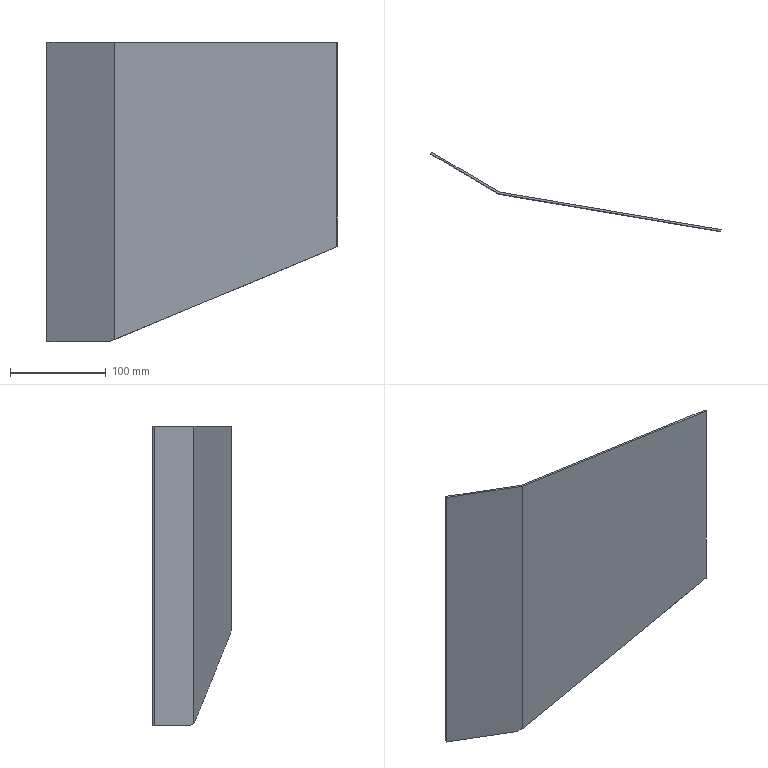Component | SolidWorks | LeftMaterialInletPlate-1 | 1 solid | 11 faces | box 303.24 x 82.86 x 313 mm | volume 174651 mm3 | plane 11
STEP:
#1=COLOUR_RGB('',0.7922,0.8196,0.9333);
#2=FILL_AREA_STYLE_COLOUR('',#1);
#3=FILL_AREA_STYLE('',(#2));
#4=SURFACE_STYLE_FILL_AREA(#3);
#5=SURFACE_SIDE_STYLE('',(#4));
#6=SURFACE_STYLE_USAGE(.BOTH.,#5);
#7=PRESENTATION_STYLE_ASSIGNMENT((#6));
#8=CARTESIAN_POINT('',(-3.729,-25.956,-0.4535));
#9=VERTEX_POINT('',#8);
#10=CARTESIAN_POINT('',(-3.731,-25.969,-0.4535));
#11=VERTEX_POINT('',#10);
#12=CARTESIAN_POINT('',(-3.667,-25.59,-0.4535));
#13=DIRECTION('',(-0.1671,-0.9859,-0.));
#14=VECTOR('',#13,39.37);
#15=LINE('',#12,#14);
#16=EDGE_CURVE('',#9,#11,#15,.T.);
#17=ORIENTED_EDGE('',*,*,#16,.F.);
#18=CARTESIAN_POINT('',(-3.543,-25.989,-0.3759));
#19=VERTEX_POINT('',#18);
#20=CARTESIAN_POINT('',(5.621,-27.645,3.443));
#21=DIRECTION('',(0.9105,-0.1645,0.3794));
#22=VECTOR('',#21,39.37);
#23=LINE('',#20,#22);
#24=EDGE_CURVE('',#9,#19,#23,.T.);
#25=ORIENTED_EDGE('',*,*,#24,.T.);
#26=CARTESIAN_POINT('',(-3.495,-26.018,-0.3543));
#27=VERTEX_POINT('',#26);
#28=CARTESIAN_POINT('',(-3.064,-26.273,-0.163));
#29=DIRECTION('',(-0.8037,0.4756,-0.3576));
#30=VECTOR('',#29,39.37);
#31=LINE('',#28,#30);
#32=EDGE_CURVE('',#27,#19,#31,.T.);
#33=ORIENTED_EDGE('',*,*,#32,.F.);
#34=CARTESIAN_POINT('',(-1.706,-26.321,0.3897));
#35=VERTEX_POINT('',#34);
#36=CARTESIAN_POINT('',(-6.771,-25.463,-1.717));
#37=DIRECTION('',(0.9122,-0.1546,0.3795));
#38=VECTOR('',#37,39.37);
#39=LINE('',#36,#38);
#40=EDGE_CURVE('',#27,#35,#39,.T.);
#41=ORIENTED_EDGE('',*,*,#40,.T.);
#42=CARTESIAN_POINT('',(5.454,-27.615,3.373));
#43=VERTEX_POINT('',#42);
#44=CARTESIAN_POINT('',(5.621,-27.645,3.443));
#45=DIRECTION('',(0.9105,-0.1645,0.3794));
#46=VECTOR('',#45,39.37);
#47=LINE('',#44,#46);
#48=EDGE_CURVE('',#35,#43,#47,.T.);
#49=ORIENTED_EDGE('',*,*,#48,.T.);
#50=CARTESIAN_POINT('',(-3.522,-26.093,-0.3603));
#51=VERTEX_POINT('',#50);
#52=CARTESIAN_POINT('',(-6.784,-25.541,-1.717));
#53=DIRECTION('',(0.9122,-0.1546,0.3795));
#54=VECTOR('',#53,39.37);
#55=LINE('',#52,#54);
#56=EDGE_CURVE('',#51,#43,#55,.T.);
#57=ORIENTED_EDGE('',*,*,#56,.F.);
#58=CARTESIAN_POINT('',(-3.101,-26.342,-0.1731));
#59=DIRECTION('',(-0.8037,0.4756,-0.3576));
#60=VECTOR('',#59,39.37);
#61=LINE('',#58,#60);
#62=EDGE_CURVE('',#51,#11,#61,.T.);
#63=ORIENTED_EDGE('',*,*,#62,.T.);
#64=EDGE_LOOP('',(#17,#25,#33,#41,#49,#57,#63));
#65=FACE_OUTER_BOUND('',#64,.T.);
#66=CARTESIAN_POINT('',(5.704,-27.178,3.445));
#67=DIRECTION('',(0.3741,-0.0634,-0.9252));
#68=DIRECTION('',(-0.8037,0.4756,-0.3576));
#69=AXIS2_PLACEMENT_3D('',#66,#67,#68);
#70=PLANE('',#69);
#71=ADVANCED_FACE('',(#65),#70,.T.);
#72=CARTESIAN_POINT('',(-3.837,-25.815,-0.4535));
#73=VERTEX_POINT('',#72);
#74=CARTESIAN_POINT('',(-5.432,-23.744,-0.4535));
#75=DIRECTION('',(-0.61,0.7924,0.));
#76=VECTOR('',#75,39.37);
#77=LINE('',#74,#76);
#78=EDGE_CURVE('',#9,#73,#77,.T.);
#79=ORIENTED_EDGE('',*,*,#78,.F.);
#80=ORIENTED_EDGE('',*,*,#16,.T.);
#81=CARTESIAN_POINT('',(-6.3,-24.449,-0.4535));
#82=VERTEX_POINT('',#81);
#83=CARTESIAN_POINT('',(-6.3,-24.449,-0.4535));
#84=DIRECTION('',(-0.8606,0.5093,0.));
#85=VECTOR('',#84,39.37);
#86=LINE('',#83,#85);
#87=EDGE_CURVE('',#11,#82,#86,.T.);
#88=ORIENTED_EDGE('',*,*,#87,.T.);
#89=CARTESIAN_POINT('',(-6.26,-24.381,-0.4535));
#90=VERTEX_POINT('',#89);
#91=CARTESIAN_POINT('',(-6.26,-24.381,-0.4535));
#92=DIRECTION('',(-0.5093,-0.8606,-0.));
#93=VECTOR('',#92,39.37);
#94=LINE('',#91,#93);
#95=EDGE_CURVE('',#90,#82,#94,.T.);
#96=ORIENTED_EDGE('',*,*,#95,.F.);
#97=CARTESIAN_POINT('',(-6.26,-24.381,-0.4535));
#98=DIRECTION('',(-0.8606,0.5093,0.));
#99=VECTOR('',#98,39.37);
#100=LINE('',#97,#99);
#101=EDGE_CURVE('',#73,#90,#100,.T.);
#102=ORIENTED_EDGE('',*,*,#101,.F.);
#103=EDGE_LOOP('',(#79,#80,#88,#96,#102));
#104=FACE_OUTER_BOUND('',#103,.T.);
#105=CARTESIAN_POINT('',(-6.26,-24.381,-0.4535));
#106=DIRECTION('',(-0.,0.,1.));
#107=DIRECTION('',(-0.5093,-0.8606,-0.));
#108=AXIS2_PLACEMENT_3D('',#105,#106,#107);
#109=PLANE('',#108);
#110=ADVANCED_FACE('',(#104),#109,.F.);
#111=CARTESIAN_POINT('',(5.638,-27.566,3.481));
#112=VERTEX_POINT('',#111);
#113=CARTESIAN_POINT('',(5.625,-27.644,3.446));
#114=VERTEX_POINT('',#113);
#115=CARTESIAN_POINT('',(4.811,-32.448,1.261));
#116=DIRECTION('',(-0.1525,-0.8997,-0.4091));
#117=VECTOR('',#116,39.37);
#118=LINE('',#115,#117);
#119=EDGE_CURVE('',#112,#114,#118,.T.);
#120=ORIENTED_EDGE('',*,*,#119,.F.);
#121=CARTESIAN_POINT('',(5.638,-27.566,11.869));
#122=VERTEX_POINT('',#121);
#123=CARTESIAN_POINT('',(5.638,-27.566,-9.784));
#124=DIRECTION('',(0.,0.,1.));
#125=VECTOR('',#124,39.37);
#126=LINE('',#123,#125);
#127=EDGE_CURVE('',#112,#122,#126,.T.);
#128=ORIENTED_EDGE('',*,*,#127,.T.);
#129=CARTESIAN_POINT('',(5.625,-27.644,11.869));
#130=VERTEX_POINT('',#129);
#131=CARTESIAN_POINT('',(5.638,-27.566,11.869));
#132=DIRECTION('',(-0.1671,-0.9859,-0.));
#133=VECTOR('',#132,39.37);
#134=LINE('',#131,#133);
#135=EDGE_CURVE('',#122,#130,#134,.T.);
#136=ORIENTED_EDGE('',*,*,#135,.T.);
#137=CARTESIAN_POINT('',(5.625,-27.644,-9.784));
#138=DIRECTION('',(0.,0.,1.));
#139=VECTOR('',#138,39.37);
#140=LINE('',#137,#139);
#141=EDGE_CURVE('',#114,#130,#140,.T.);
#142=ORIENTED_EDGE('',*,*,#141,.F.);
#143=EDGE_LOOP('',(#120,#128,#136,#142));
#144=FACE_OUTER_BOUND('',#143,.T.);
#145=CARTESIAN_POINT('',(5.638,-27.566,-9.784));
#146=DIRECTION('',(-0.9859,0.1671,0.));
#147=DIRECTION('',(0.1671,0.9859,0.));
#148=AXIS2_PLACEMENT_3D('',#145,#146,#147);
#149=PLANE('',#148);
#150=ADVANCED_FACE('',(#144),#149,.F.);
#151=ORIENTED_EDGE('',*,*,#127,.F.);
#152=CARTESIAN_POINT('',(-6.795,-25.459,-1.752));
#153=DIRECTION('',(0.9106,-0.1543,0.3833));
#154=VECTOR('',#153,39.37);
#155=LINE('',#152,#154);
#156=EDGE_CURVE('',#35,#112,#155,.T.);
#157=ORIENTED_EDGE('',*,*,#156,.F.);
#158=ORIENTED_EDGE('',*,*,#40,.F.);
#159=CARTESIAN_POINT('',(-3.495,-26.018,11.869));
#160=VERTEX_POINT('',#159);
#161=CARTESIAN_POINT('',(-3.495,-26.018,1.063));
#162=DIRECTION('',(0.,-0.,-1.));
#163=VECTOR('',#162,39.37);
#164=LINE('',#161,#163);
#165=EDGE_CURVE('',#160,#27,#164,.T.);
#166=ORIENTED_EDGE('',*,*,#165,.F.);
#167=CARTESIAN_POINT('',(-3.509,-26.016,11.869));
#168=DIRECTION('',(0.9859,-0.1671,-0.));
#169=VECTOR('',#168,39.37);
#170=LINE('',#167,#169);
#171=EDGE_CURVE('',#160,#122,#170,.T.);
#172=ORIENTED_EDGE('',*,*,#171,.T.);
#173=EDGE_LOOP('',(#151,#157,#158,#166,#172));
#174=FACE_OUTER_BOUND('',#173,.T.);
#175=CARTESIAN_POINT('',(-3.509,-26.016,-9.784));
#176=DIRECTION('',(-0.1671,-0.9859,-0.));
#177=DIRECTION('',(-0.9859,0.1671,0.));
#178=AXIS2_PLACEMENT_3D('',#175,#176,#177);
#179=PLANE('',#178);
#180=ADVANCED_FACE('',(#174),#179,.F.);
#181=ORIENTED_EDGE('',*,*,#32,.T.);
#182=CARTESIAN_POINT('',(-3.205,-26.19,-0.2869));
#183=DIRECTION('',(-0.8393,0.4967,-0.2211));
#184=VECTOR('',#183,39.37);
#185=LINE('',#182,#184);
#186=EDGE_CURVE('',#19,#73,#185,.T.);
#187=ORIENTED_EDGE('',*,*,#186,.T.);
#188=ORIENTED_EDGE('',*,*,#101,.T.);
#189=CARTESIAN_POINT('',(-6.26,-24.381,11.869));
#190=VERTEX_POINT('',#189);
#191=CARTESIAN_POINT('',(-6.26,-24.381,-0.4535));
#192=DIRECTION('',(0.,-0.,1.));
#193=VECTOR('',#192,39.37);
#194=LINE('',#191,#193);
#195=EDGE_CURVE('',#90,#190,#194,.T.);
#196=ORIENTED_EDGE('',*,*,#195,.T.);
#197=CARTESIAN_POINT('',(-6.26,-24.381,11.869));
#198=DIRECTION('',(0.8606,-0.5093,-0.));
#199=VECTOR('',#198,39.37);
#200=LINE('',#197,#199);
#201=EDGE_CURVE('',#190,#160,#200,.T.);
#202=ORIENTED_EDGE('',*,*,#201,.T.);
#203=ORIENTED_EDGE('',*,*,#165,.T.);
#204=EDGE_LOOP('',(#181,#187,#188,#196,#202,#203));
#205=FACE_OUTER_BOUND('',#204,.T.);
#206=CARTESIAN_POINT('',(-3.468,-26.034,1.063));
#207=DIRECTION('',(0.5093,0.8606,0.));
#208=DIRECTION('',(0.8606,-0.5093,-0.));
#209=AXIS2_PLACEMENT_3D('',#206,#207,#208);
#210=PLANE('',#209);
#211=ADVANCED_FACE('',(#205),#210,.T.);
#212=ORIENTED_EDGE('',*,*,#56,.T.);
#213=CARTESIAN_POINT('',(-6.796,-25.539,-1.782));
#214=DIRECTION('',(0.9106,-0.1543,0.3833));
#215=VECTOR('',#214,39.37);
#216=LINE('',#213,#215);
#217=EDGE_CURVE('',#43,#114,#216,.T.);
#218=ORIENTED_EDGE('',*,*,#217,.T.);
#219=ORIENTED_EDGE('',*,*,#141,.T.);
#220=CARTESIAN_POINT('',(-3.522,-26.093,11.869));
#221=VERTEX_POINT('',#220);
#222=CARTESIAN_POINT('',(-3.522,-26.093,11.869));
#223=DIRECTION('',(0.9859,-0.1671,-0.));
#224=VECTOR('',#223,39.37);
#225=LINE('',#222,#224);
#226=EDGE_CURVE('',#221,#130,#225,.T.);
#227=ORIENTED_EDGE('',*,*,#226,.F.);
#228=CARTESIAN_POINT('',(-3.522,-26.093,-0.4535));
#229=DIRECTION('',(-0.,0.,-1.));
#230=VECTOR('',#229,39.37);
#231=LINE('',#228,#230);
#232=EDGE_CURVE('',#221,#51,#231,.T.);
#233=ORIENTED_EDGE('',*,*,#232,.T.);
#234=EDGE_LOOP('',(#212,#218,#219,#227,#233));
#235=FACE_OUTER_BOUND('',#234,.T.);
#236=CARTESIAN_POINT('',(-3.522,-26.093,-9.784));
#237=DIRECTION('',(-0.1671,-0.9859,-0.));
#238=DIRECTION('',(-0.9859,0.1671,0.));
#239=AXIS2_PLACEMENT_3D('',#236,#237,#238);
#240=PLANE('',#239);
#241=ADVANCED_FACE('',(#235),#240,.T.);
#242=ORIENTED_EDGE('',*,*,#62,.F.);
#243=ORIENTED_EDGE('',*,*,#232,.F.);
#244=CARTESIAN_POINT('',(-6.3,-24.449,11.869));
#245=VERTEX_POINT('',#244);
#246=CARTESIAN_POINT('',(-6.3,-24.449,11.869));
#247=DIRECTION('',(0.8606,-0.5093,-0.));
#248=VECTOR('',#247,39.37);
#249=LINE('',#246,#248);
#250=EDGE_CURVE('',#245,#221,#249,.T.);
#251=ORIENTED_EDGE('',*,*,#250,.F.);
#252=CARTESIAN_POINT('',(-6.3,-24.449,-0.4535));
#253=DIRECTION('',(0.,-0.,1.));
#254=VECTOR('',#253,39.37);
#255=LINE('',#252,#254);
#256=EDGE_CURVE('',#82,#245,#255,.T.);
#257=ORIENTED_EDGE('',*,*,#256,.F.);
#258=ORIENTED_EDGE('',*,*,#87,.F.);
#259=EDGE_LOOP('',(#242,#243,#251,#257,#258));
#260=FACE_OUTER_BOUND('',#259,.T.);
#261=CARTESIAN_POINT('',(-3.509,-26.101,1.063));
#262=DIRECTION('',(0.5093,0.8606,0.));
#263=DIRECTION('',(0.8606,-0.5093,-0.));
#264=AXIS2_PLACEMENT_3D('',#261,#262,#263);
#265=PLANE('',#264);
#266=ADVANCED_FACE('',(#260),#265,.F.);
#267=ORIENTED_EDGE('',*,*,#256,.T.);
#268=CARTESIAN_POINT('',(-6.26,-24.381,11.869));
#269=DIRECTION('',(-0.5093,-0.8606,-0.));
#270=VECTOR('',#269,39.37);
#271=LINE('',#268,#270);
#272=EDGE_CURVE('',#190,#245,#271,.T.);
#273=ORIENTED_EDGE('',*,*,#272,.F.);
#274=ORIENTED_EDGE('',*,*,#195,.F.);
#275=ORIENTED_EDGE('',*,*,#95,.T.);
#276=EDGE_LOOP('',(#267,#273,#274,#275));
#277=FACE_OUTER_BOUND('',#276,.T.);
#278=CARTESIAN_POINT('',(-6.26,-24.381,-0.4535));
#279=DIRECTION('',(0.8606,-0.5093,-0.));
#280=DIRECTION('',(-0.,0.,-1.));
#281=AXIS2_PLACEMENT_3D('',#278,#279,#280);
#282=PLANE('',#281);
#283=ADVANCED_FACE('',(#277),#282,.F.);
#284=ORIENTED_EDGE('',*,*,#171,.F.);
#285=ORIENTED_EDGE('',*,*,#201,.F.);
#286=ORIENTED_EDGE('',*,*,#272,.T.);
#287=ORIENTED_EDGE('',*,*,#250,.T.);
#288=ORIENTED_EDGE('',*,*,#226,.T.);
#289=ORIENTED_EDGE('',*,*,#135,.F.);
#290=EDGE_LOOP('',(#284,#285,#286,#287,#288,#289));
#291=FACE_OUTER_BOUND('',#290,.T.);
#292=CARTESIAN_POINT('',(-6.26,-24.381,11.869));
#293=DIRECTION('',(0.,-0.,-1.));
#294=DIRECTION('',(0.5093,0.8606,0.));
#295=AXIS2_PLACEMENT_3D('',#292,#293,#294);
#296=PLANE('',#295);
#297=ADVANCED_FACE('',(#291),#296,.F.);
#298=ORIENTED_EDGE('',*,*,#24,.F.);
#299=ORIENTED_EDGE('',*,*,#78,.T.);
#300=ORIENTED_EDGE('',*,*,#186,.F.);
#301=EDGE_LOOP('',(#298,#299,#300));
#302=FACE_OUTER_BOUND('',#301,.T.);
#303=CARTESIAN_POINT('',(-2.992,-25.704,-0.003039));
#304=DIRECTION('',(0.4131,0.318,-0.8534));
#305=DIRECTION('',(0.443,0.7485,0.4934));
#306=AXIS2_PLACEMENT_3D('',#303,#304,#305);
#307=PLANE('',#306);
#308=ADVANCED_FACE('',(#302),#307,.T.);
#309=ORIENTED_EDGE('',*,*,#119,.T.);
#310=ORIENTED_EDGE('',*,*,#217,.F.);
#311=ORIENTED_EDGE('',*,*,#48,.F.);
#312=ORIENTED_EDGE('',*,*,#156,.T.);
#313=EDGE_LOOP('',(#309,#310,#311,#312));
#314=FACE_OUTER_BOUND('',#313,.T.);
#315=CARTESIAN_POINT('',(-2.992,-25.704,-0.003039));
#316=DIRECTION('',(0.4131,0.318,-0.8534));
#317=DIRECTION('',(0.443,0.7485,0.4934));
#318=AXIS2_PLACEMENT_3D('',#315,#316,#317);
#319=PLANE('',#318);
#320=ADVANCED_FACE('',(#314),#319,.T.);
#321=CLOSED_SHELL('',(#71,#110,#150,#180,#211,#241,#266,#283,#297,#308,#320));
#322=MANIFOLD_SOLID_BREP('',#321);
#323=STYLED_ITEM('',(#7),#322);
#324=PRESENTATION_LAYER_ASSIGNMENT('','',(#323));
#325=CARTESIAN_POINT('',(0.,0.,0.));
#326=DIRECTION('',(0.,0.,1.));
#327=DIRECTION('',(1.,0.,0.));
#328=AXIS2_PLACEMENT_3D('',#325,#326,#327);
#329=(LENGTH_UNIT()NAMED_UNIT(*)SI_UNIT($,.METRE.));
#330=LENGTH_MEASURE_WITH_UNIT(LENGTH_MEASURE(0.0254),#329);
#331=DIMENSIONAL_EXPONENTS(1.,0.,0.,0.,0.,0.,0.);
#332=(CONVERSION_BASED_UNIT('',#330)LENGTH_UNIT()NAMED_UNIT(#331));
#333=UNCERTAINTY_MEASURE_WITH_UNIT(LENGTH_MEASURE(0.00001),#332,'','');
#334=(NAMED_UNIT(*)PLANE_ANGLE_UNIT()SI_UNIT($,.RADIAN.));
#335=(NAMED_UNIT(*)SI_UNIT($,.STERADIAN.)SOLID_ANGLE_UNIT());
#336=(GEOMETRIC_REPRESENTATION_CONTEXT(3)GLOBAL_UNCERTAINTY_ASSIGNED_CONTEXT((#333))GLOBAL_UNIT_ASSIGNED_CONTEXT((#332,#334,#335))REPRESENTATION_CONTEXT('',''));
#337=ADVANCED_BREP_SHAPE_REPRESENTATION('',(#322,#328),#336);
#338=(LENGTH_UNIT()NAMED_UNIT(*)SI_UNIT($,.METRE.));
#339=LENGTH_MEASURE_WITH_UNIT(LENGTH_MEASURE(0.0254),#338);
#340=DIMENSIONAL_EXPONENTS(1.,0.,0.,0.,0.,0.,0.);
#341=(CONVERSION_BASED_UNIT('',#339)LENGTH_UNIT()NAMED_UNIT(#340));
#342=UNCERTAINTY_MEASURE_WITH_UNIT(LENGTH_MEASURE(0.00001),#341,'','');
#343=(NAMED_UNIT(*)PLANE_ANGLE_UNIT()SI_UNIT($,.RADIAN.));
#344=(NAMED_UNIT(*)SI_UNIT($,.STERADIAN.)SOLID_ANGLE_UNIT());
#345=(GEOMETRIC_REPRESENTATION_CONTEXT(3)GLOBAL_UNCERTAINTY_ASSIGNED_CONTEXT((#342))GLOBAL_UNIT_ASSIGNED_CONTEXT((#341,#343,#344))REPRESENTATION_CONTEXT('',''));
#346=MECHANICAL_DESIGN_GEOMETRIC_PRESENTATION_REPRESENTATION('',(#323),#345);